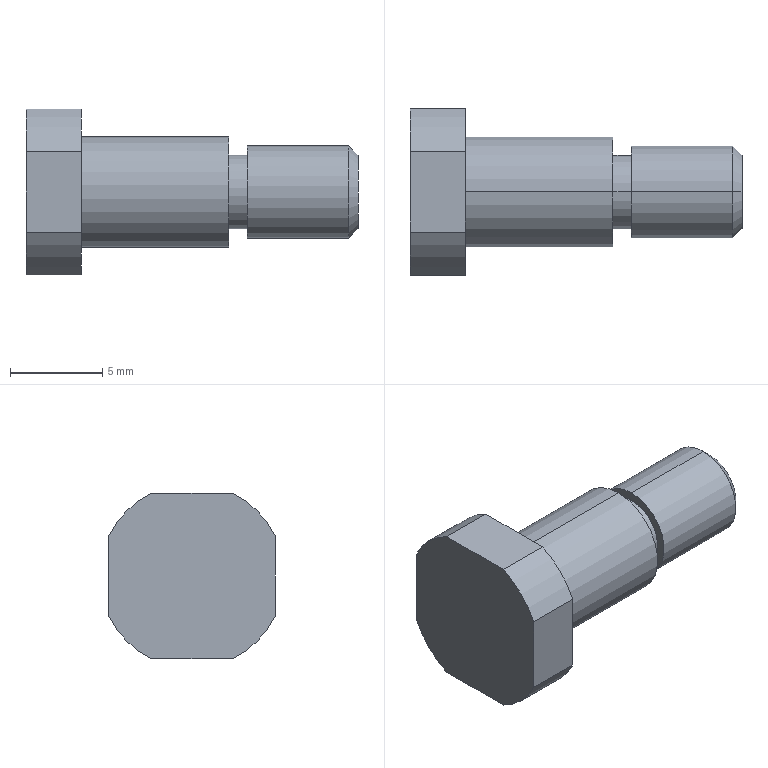Component | SolidWorks | A51-3 | 1 solid | 21 faces | box 18 x 9 x 9 mm | volume 573 mm3 | cylinder 10 | plane 9 | cone 2 | commonest cylinder face diameters 10 x4 5 x2 4 x2 6 x2 | material SUS304
build123d program:
from build123d import *

# Parameters (mm, degrees)
SKETCH12_R           = 5
BOSS_EXTRUDE3_DEPTH  = 3
SKETCH13_R           = 3
BOSS_EXTRUDE4_DEPTH  = 8
SKETCH14_R           = 2
BOSS_EXTRUDE5_DEPTH  = 1
SKETCH15_R           = 2.5
BOSS_EXTRUDE6_DEPTH  = 6
CHAMFER4_SIZE        = 0.5
SKETCH16_OUTSIDE_W   = 16.578
SKETCH16_OUTSIDE_H   = 16.578
SKETCH16_OUTSIDE_W_2 = 9
SKETCH16_OUTSIDE_H_2 = 9
CUT_EXTRUDE1_DEPTH   = 20.339


with BuildPart() as part:
    # Sketch12 → Boss-Extrude3 (new body)
    with BuildSketch(Plane(origin=(0, 0, 0), x_dir=(0, 0, -1), z_dir=(1, 0, 0))):
        Circle(SKETCH12_R)
    extrude(amount=BOSS_EXTRUDE3_DEPTH)

    # Sketch13 → Boss-Extrude4 (add)
    with BuildSketch(Plane.ZY):
        Circle(SKETCH13_R)
    extrude(amount=BOSS_EXTRUDE4_DEPTH)

    # Sketch14 → Boss-Extrude5 (add)
    with BuildSketch(Plane.ZY.offset(8)):
        Circle(SKETCH14_R)
    extrude(amount=BOSS_EXTRUDE5_DEPTH)

    # Sketch15 → Boss-Extrude6 (add)
    with BuildSketch(Plane.ZY.offset(9)):
        Circle(SKETCH15_R)
    extrude(amount=BOSS_EXTRUDE6_DEPTH)

    # Chamfer4
    chamfer4_edges = [part.edges().sort_by_distance(p)[0] for p in [
        (-15, 0, -2.5),
    ]]
    chamfer(chamfer4_edges, length=CHAMFER4_SIZE)

    # Sketch16 outside → Cut-Extrude1 (cut, through all)
    with BuildSketch(Plane(origin=(3, 0, 0), x_dir=(0, 0, -1), z_dir=(1, 0, 0))):
        Rectangle(SKETCH16_OUTSIDE_W, SKETCH16_OUTSIDE_H)
        Rectangle(SKETCH16_OUTSIDE_W_2, SKETCH16_OUTSIDE_H_2, mode=Mode.SUBTRACT)
    extrude(amount=-CUT_EXTRUDE1_DEPTH, mode=Mode.SUBTRACT)


solid = part.part

# Placed as in the assembly
solid = solid.moved(Location((-25.351, 25.864, 5), (-180, 0, 180)))
STEP:
#1=CARTESIAN_POINT('',(-0.4075,1.018,0.1181));
#2=VERTEX_POINT('',#1);
#3=CARTESIAN_POINT('',(-0.4075,1.018,0.2756));
#4=VERTEX_POINT('',#3);
#5=CARTESIAN_POINT('',(-0.4075,1.018,0.1969));
#6=DIRECTION('',(1.,0.,0.));
#7=DIRECTION('',(0.,0.,-1.));
#8=AXIS2_PLACEMENT_3D('',#5,#6,#7);
#9=CIRCLE('',#8,0.07874);
#10=EDGE_CURVE('',#2,#4,#9,.T.);
#11=ORIENTED_EDGE('',*,*,#10,.F.);
#12=CARTESIAN_POINT('',(-0.4272,1.018,0.09843));
#13=VERTEX_POINT('',#12);
#14=CARTESIAN_POINT('',(-0.4075,1.018,0.1181));
#15=DIRECTION('',(-0.7071,0.,-0.7071));
#16=VECTOR('',#15,39.37);
#17=LINE('',#14,#16);
#18=EDGE_CURVE('',#2,#13,#17,.T.);
#19=ORIENTED_EDGE('',*,*,#18,.T.);
#20=CARTESIAN_POINT('',(-0.4272,1.018,0.2953));
#21=VERTEX_POINT('',#20);
#22=CARTESIAN_POINT('',(-0.4272,1.018,0.1969));
#23=DIRECTION('',(-1.,-0.,-0.));
#24=DIRECTION('',(0.,0.,-1.));
#25=AXIS2_PLACEMENT_3D('',#22,#23,#24);
#26=CIRCLE('',#25,0.09843);
#27=EDGE_CURVE('',#21,#13,#26,.T.);
#28=ORIENTED_EDGE('',*,*,#27,.F.);
#29=CARTESIAN_POINT('',(-0.4075,1.018,0.2756));
#30=DIRECTION('',(-0.7071,-0.,0.7071));
#31=VECTOR('',#30,39.37);
#32=LINE('',#29,#31);
#33=EDGE_CURVE('',#4,#21,#32,.T.);
#34=ORIENTED_EDGE('',*,*,#33,.F.);
#35=EDGE_LOOP('',(#11,#19,#28,#34));
#36=FACE_OUTER_BOUND('',#35,.T.);
#37=CARTESIAN_POINT('',(-0.4075,1.018,0.1969));
#38=DIRECTION('',(-1.,-0.,-0.));
#39=DIRECTION('',(0.,0.,1.));
#40=AXIS2_PLACEMENT_3D('',#37,#38,#39);
#41=CONICAL_SURFACE('',#40,0.07874,0.7854);
#42=ADVANCED_FACE('',(#36),#41,.T.);
#43=ORIENTED_EDGE('',*,*,#27,.T.);
#44=CARTESIAN_POINT('',(-0.6437,1.018,0.09843));
#45=VERTEX_POINT('',#44);
#46=CARTESIAN_POINT('',(-0.4075,1.018,0.09843));
#47=DIRECTION('',(-1.,-0.,-0.));
#48=VECTOR('',#47,39.37);
#49=LINE('',#46,#48);
#50=EDGE_CURVE('',#13,#45,#49,.T.);
#51=ORIENTED_EDGE('',*,*,#50,.T.);
#52=CARTESIAN_POINT('',(-0.6437,1.018,0.2953));
#53=VERTEX_POINT('',#52);
#54=CARTESIAN_POINT('',(-0.6437,1.018,0.1969));
#55=DIRECTION('',(1.,0.,0.));
#56=DIRECTION('',(0.,0.,-1.));
#57=AXIS2_PLACEMENT_3D('',#54,#55,#56);
#58=CIRCLE('',#57,0.09843);
#59=EDGE_CURVE('',#45,#53,#58,.T.);
#60=ORIENTED_EDGE('',*,*,#59,.T.);
#61=CARTESIAN_POINT('',(-0.4075,1.018,0.2953));
#62=DIRECTION('',(-1.,-0.,-0.));
#63=VECTOR('',#62,39.37);
#64=LINE('',#61,#63);
#65=EDGE_CURVE('',#21,#53,#64,.T.);
#66=ORIENTED_EDGE('',*,*,#65,.F.);
#67=EDGE_LOOP('',(#43,#51,#60,#66));
#68=FACE_OUTER_BOUND('',#67,.T.);
#69=CARTESIAN_POINT('',(-0.4075,1.018,0.1969));
#70=DIRECTION('',(-1.,-0.,-0.));
#71=DIRECTION('',(0.,0.,1.));
#72=AXIS2_PLACEMENT_3D('',#69,#70,#71);
#73=CYLINDRICAL_SURFACE('',#72,0.09843);
#74=ADVANCED_FACE('',(#68),#73,.T.);
#75=CARTESIAN_POINT('',(-0.6437,1.018,0.1181));
#76=VERTEX_POINT('',#75);
#77=CARTESIAN_POINT('',(-0.6437,1.018,0.2756));
#78=VERTEX_POINT('',#77);
#79=CARTESIAN_POINT('',(-0.6437,1.018,0.1969));
#80=DIRECTION('',(1.,0.,0.));
#81=DIRECTION('',(0.,0.,-1.));
#82=AXIS2_PLACEMENT_3D('',#79,#80,#81);
#83=CIRCLE('',#82,0.07874);
#84=EDGE_CURVE('',#76,#78,#83,.T.);
#85=ORIENTED_EDGE('',*,*,#84,.F.);
#86=CARTESIAN_POINT('',(-0.6831,1.018,0.1181));
#87=VERTEX_POINT('',#86);
#88=CARTESIAN_POINT('',(-0.6437,1.018,0.1181));
#89=DIRECTION('',(-1.,-0.,-0.));
#90=VECTOR('',#89,39.37);
#91=LINE('',#88,#90);
#92=EDGE_CURVE('',#76,#87,#91,.T.);
#93=ORIENTED_EDGE('',*,*,#92,.T.);
#94=CARTESIAN_POINT('',(-0.6831,1.018,0.2756));
#95=VERTEX_POINT('',#94);
#96=CARTESIAN_POINT('',(-0.6831,1.018,0.1969));
#97=DIRECTION('',(1.,0.,0.));
#98=DIRECTION('',(0.,0.,-1.));
#99=AXIS2_PLACEMENT_3D('',#96,#97,#98);
#100=CIRCLE('',#99,0.07874);
#101=EDGE_CURVE('',#87,#95,#100,.T.);
#102=ORIENTED_EDGE('',*,*,#101,.T.);
#103=CARTESIAN_POINT('',(-0.6437,1.018,0.2756));
#104=DIRECTION('',(-1.,-0.,-0.));
#105=VECTOR('',#104,39.37);
#106=LINE('',#103,#105);
#107=EDGE_CURVE('',#78,#95,#106,.T.);
#108=ORIENTED_EDGE('',*,*,#107,.F.);
#109=EDGE_LOOP('',(#85,#93,#102,#108));
#110=FACE_OUTER_BOUND('',#109,.T.);
#111=CARTESIAN_POINT('',(-0.6437,1.018,0.1969));
#112=DIRECTION('',(-1.,-0.,-0.));
#113=DIRECTION('',(0.,0.,1.));
#114=AXIS2_PLACEMENT_3D('',#111,#112,#113);
#115=CYLINDRICAL_SURFACE('',#114,0.07874);
#116=ADVANCED_FACE('',(#110),#115,.T.);
#117=CARTESIAN_POINT('',(-0.6831,1.018,0.07874));
#118=VERTEX_POINT('',#117);
#119=CARTESIAN_POINT('',(-0.6831,1.018,0.315));
#120=VERTEX_POINT('',#119);
#121=CARTESIAN_POINT('',(-0.6831,1.018,0.1969));
#122=DIRECTION('',(1.,0.,0.));
#123=DIRECTION('',(0.,0.,-1.));
#124=AXIS2_PLACEMENT_3D('',#121,#122,#123);
#125=CIRCLE('',#124,0.1181);
#126=EDGE_CURVE('',#118,#120,#125,.T.);
#127=ORIENTED_EDGE('',*,*,#126,.F.);
#128=CARTESIAN_POINT('',(-0.9981,1.018,0.07874));
#129=VERTEX_POINT('',#128);
#130=CARTESIAN_POINT('',(-0.6831,1.018,0.07874));
#131=DIRECTION('',(-1.,-0.,-0.));
#132=VECTOR('',#131,39.37);
#133=LINE('',#130,#132);
#134=EDGE_CURVE('',#118,#129,#133,.T.);
#135=ORIENTED_EDGE('',*,*,#134,.T.);
#136=CARTESIAN_POINT('',(-0.9981,1.018,0.315));
#137=VERTEX_POINT('',#136);
#138=CARTESIAN_POINT('',(-0.9981,1.018,0.1969));
#139=DIRECTION('',(1.,0.,0.));
#140=DIRECTION('',(0.,0.,-1.));
#141=AXIS2_PLACEMENT_3D('',#138,#139,#140);
#142=CIRCLE('',#141,0.1181);
#143=EDGE_CURVE('',#129,#137,#142,.T.);
#144=ORIENTED_EDGE('',*,*,#143,.T.);
#145=CARTESIAN_POINT('',(-0.6831,1.018,0.315));
#146=DIRECTION('',(-1.,-0.,-0.));
#147=VECTOR('',#146,39.37);
#148=LINE('',#145,#147);
#149=EDGE_CURVE('',#120,#137,#148,.T.);
#150=ORIENTED_EDGE('',*,*,#149,.F.);
#151=EDGE_LOOP('',(#127,#135,#144,#150));
#152=FACE_OUTER_BOUND('',#151,.T.);
#153=CARTESIAN_POINT('',(-0.6831,1.018,0.1969));
#154=DIRECTION('',(-1.,-0.,-0.));
#155=DIRECTION('',(0.,0.,1.));
#156=AXIS2_PLACEMENT_3D('',#153,#154,#155);
#157=CYLINDRICAL_SURFACE('',#156,0.1181);
#158=ADVANCED_FACE('',(#152),#157,.T.);
#159=CARTESIAN_POINT('',(-1.116,0.9325,0.374));
#160=VERTEX_POINT('',#159);
#161=CARTESIAN_POINT('',(-0.9981,0.9325,0.374));
#162=VERTEX_POINT('',#161);
#163=CARTESIAN_POINT('',(-1.116,0.9325,0.374));
#164=DIRECTION('',(1.,0.,0.));
#165=VECTOR('',#164,39.37);
#166=LINE('',#163,#165);
#167=EDGE_CURVE('',#160,#162,#166,.T.);
#168=ORIENTED_EDGE('',*,*,#167,.F.);
#169=CARTESIAN_POINT('',(-1.116,0.8411,0.2827));
#170=VERTEX_POINT('',#169);
#171=CARTESIAN_POINT('',(-1.116,1.018,0.1969));
#172=DIRECTION('',(-1.,-0.,-0.));
#173=DIRECTION('',(0.,0.,1.));
#174=AXIS2_PLACEMENT_3D('',#171,#172,#173);
#175=CIRCLE('',#174,0.1969);
#176=EDGE_CURVE('',#170,#160,#175,.T.);
#177=ORIENTED_EDGE('',*,*,#176,.F.);
#178=CARTESIAN_POINT('',(-0.9981,0.8411,0.2827));
#179=VERTEX_POINT('',#178);
#180=CARTESIAN_POINT('',(-1.116,0.8411,0.2827));
#181=DIRECTION('',(-1.,-0.,-0.));
#182=VECTOR('',#181,39.37);
#183=LINE('',#180,#182);
#184=EDGE_CURVE('',#179,#170,#183,.T.);
#185=ORIENTED_EDGE('',*,*,#184,.F.);
#186=CARTESIAN_POINT('',(-0.9981,1.018,0.1969));
#187=DIRECTION('',(-1.,-0.,-0.));
#188=DIRECTION('',(0.,0.,1.));
#189=AXIS2_PLACEMENT_3D('',#186,#187,#188);
#190=CIRCLE('',#189,0.1969);
#191=EDGE_CURVE('',#179,#162,#190,.T.);
#192=ORIENTED_EDGE('',*,*,#191,.T.);
#193=EDGE_LOOP('',(#168,#177,#185,#192));
#194=FACE_OUTER_BOUND('',#193,.T.);
#195=CARTESIAN_POINT('',(-1.116,1.018,0.1969));
#196=DIRECTION('',(1.,0.,0.));
#197=DIRECTION('',(0.,0.,-1.));
#198=AXIS2_PLACEMENT_3D('',#195,#196,#197);
#199=CYLINDRICAL_SURFACE('',#198,0.1969);
#200=ADVANCED_FACE('',(#194),#199,.T.);
#201=CARTESIAN_POINT('',(-0.9981,1.104,0.374));
#202=VERTEX_POINT('',#201);
#203=CARTESIAN_POINT('',(-1.116,1.104,0.374));
#204=VERTEX_POINT('',#203);
#205=CARTESIAN_POINT('',(-1.116,1.104,0.374));
#206=DIRECTION('',(-1.,-0.,-0.));
#207=VECTOR('',#206,39.37);
#208=LINE('',#205,#207);
#209=EDGE_CURVE('',#202,#204,#208,.T.);
#210=ORIENTED_EDGE('',*,*,#209,.F.);
#211=CARTESIAN_POINT('',(-0.9981,1.195,0.2827));
#212=VERTEX_POINT('',#211);
#213=CARTESIAN_POINT('',(-0.9981,1.018,0.1969));
#214=DIRECTION('',(-1.,-0.,-0.));
#215=DIRECTION('',(0.,0.,1.));
#216=AXIS2_PLACEMENT_3D('',#213,#214,#215);
#217=CIRCLE('',#216,0.1969);
#218=EDGE_CURVE('',#202,#212,#217,.T.);
#219=ORIENTED_EDGE('',*,*,#218,.T.);
#220=CARTESIAN_POINT('',(-1.116,1.195,0.2827));
#221=VERTEX_POINT('',#220);
#222=CARTESIAN_POINT('',(-1.116,1.195,0.2827));
#223=DIRECTION('',(1.,0.,0.));
#224=VECTOR('',#223,39.37);
#225=LINE('',#222,#224);
#226=EDGE_CURVE('',#221,#212,#225,.T.);
#227=ORIENTED_EDGE('',*,*,#226,.F.);
#228=CARTESIAN_POINT('',(-1.116,1.018,0.1969));
#229=DIRECTION('',(-1.,-0.,-0.));
#230=DIRECTION('',(0.,0.,1.));
#231=AXIS2_PLACEMENT_3D('',#228,#229,#230);
#232=CIRCLE('',#231,0.1969);
#233=EDGE_CURVE('',#204,#221,#232,.T.);
#234=ORIENTED_EDGE('',*,*,#233,.F.);
#235=EDGE_LOOP('',(#210,#219,#227,#234));
#236=FACE_OUTER_BOUND('',#235,.T.);
#237=CARTESIAN_POINT('',(-1.116,1.018,0.1969));
#238=DIRECTION('',(1.,0.,0.));
#239=DIRECTION('',(0.,0.,-1.));
#240=AXIS2_PLACEMENT_3D('',#237,#238,#239);
#241=CYLINDRICAL_SURFACE('',#240,0.1969);
#242=ADVANCED_FACE('',(#236),#241,.T.);
#243=CARTESIAN_POINT('',(-1.116,0.8411,0.111));
#244=VERTEX_POINT('',#243);
#245=CARTESIAN_POINT('',(-0.9981,0.8411,0.111));
#246=VERTEX_POINT('',#245);
#247=CARTESIAN_POINT('',(-1.116,0.8411,0.111));
#248=DIRECTION('',(1.,0.,0.));
#249=VECTOR('',#248,39.37);
#250=LINE('',#247,#249);
#251=EDGE_CURVE('',#244,#246,#250,.T.);
#252=ORIENTED_EDGE('',*,*,#251,.F.);
#253=CARTESIAN_POINT('',(-1.116,0.9325,0.01969));
#254=VERTEX_POINT('',#253);
#255=CARTESIAN_POINT('',(-1.116,1.018,0.1969));
#256=DIRECTION('',(-1.,-0.,-0.));
#257=DIRECTION('',(0.,0.,1.));
#258=AXIS2_PLACEMENT_3D('',#255,#256,#257);
#259=CIRCLE('',#258,0.1969);
#260=EDGE_CURVE('',#254,#244,#259,.T.);
#261=ORIENTED_EDGE('',*,*,#260,.F.);
#262=CARTESIAN_POINT('',(-0.9981,0.9325,0.01969));
#263=VERTEX_POINT('',#262);
#264=CARTESIAN_POINT('',(-1.116,0.9325,0.01969));
#265=DIRECTION('',(-1.,-0.,-0.));
#266=VECTOR('',#265,39.37);
#267=LINE('',#264,#266);
#268=EDGE_CURVE('',#263,#254,#267,.T.);
#269=ORIENTED_EDGE('',*,*,#268,.F.);
#270=CARTESIAN_POINT('',(-0.9981,1.018,0.1969));
#271=DIRECTION('',(-1.,-0.,-0.));
#272=DIRECTION('',(0.,0.,1.));
#273=AXIS2_PLACEMENT_3D('',#270,#271,#272);
#274=CIRCLE('',#273,0.1969);
#275=EDGE_CURVE('',#263,#246,#274,.T.);
#276=ORIENTED_EDGE('',*,*,#275,.T.);
#277=EDGE_LOOP('',(#252,#261,#269,#276));
#278=FACE_OUTER_BOUND('',#277,.T.);
#279=CARTESIAN_POINT('',(-1.116,1.018,0.1969));
#280=DIRECTION('',(1.,0.,0.));
#281=DIRECTION('',(0.,0.,-1.));
#282=AXIS2_PLACEMENT_3D('',#279,#280,#281);
#283=CYLINDRICAL_SURFACE('',#282,0.1969);
#284=ADVANCED_FACE('',(#278),#283,.T.);
#285=CARTESIAN_POINT('',(-1.116,1.104,0.01969));
#286=VERTEX_POINT('',#285);
#287=CARTESIAN_POINT('',(-0.9981,1.104,0.01969));
#288=VERTEX_POINT('',#287);
#289=CARTESIAN_POINT('',(-1.116,1.104,0.01969));
#290=DIRECTION('',(1.,0.,0.));
#291=VECTOR('',#290,39.37);
#292=LINE('',#289,#291);
#293=EDGE_CURVE('',#286,#288,#292,.T.);
#294=ORIENTED_EDGE('',*,*,#293,.F.);
#295=CARTESIAN_POINT('',(-1.116,1.195,0.111));
#296=VERTEX_POINT('',#295);
#297=CARTESIAN_POINT('',(-1.116,1.018,0.1969));
#298=DIRECTION('',(-1.,-0.,-0.));
#299=DIRECTION('',(0.,0.,1.));
#300=AXIS2_PLACEMENT_3D('',#297,#298,#299);
#301=CIRCLE('',#300,0.1969);
#302=EDGE_CURVE('',#296,#286,#301,.T.);
#303=ORIENTED_EDGE('',*,*,#302,.F.);
#304=CARTESIAN_POINT('',(-0.9981,1.195,0.111));
#305=VERTEX_POINT('',#304);
#306=CARTESIAN_POINT('',(-1.116,1.195,0.111));
#307=DIRECTION('',(-1.,-0.,-0.));
#308=VECTOR('',#307,39.37);
#309=LINE('',#306,#308);
#310=EDGE_CURVE('',#305,#296,#309,.T.);
#311=ORIENTED_EDGE('',*,*,#310,.F.);
#312=CARTESIAN_POINT('',(-0.9981,1.018,0.1969));
#313=DIRECTION('',(-1.,-0.,-0.));
#314=DIRECTION('',(0.,0.,1.));
#315=AXIS2_PLACEMENT_3D('',#312,#313,#314);
#316=CIRCLE('',#315,0.1969);
#317=EDGE_CURVE('',#305,#288,#316,.T.);
#318=ORIENTED_EDGE('',*,*,#317,.T.);
#319=EDGE_LOOP('',(#294,#303,#311,#318));
#320=FACE_OUTER_BOUND('',#319,.T.);
#321=CARTESIAN_POINT('',(-1.116,1.018,0.1969));
#322=DIRECTION('',(1.,0.,0.));
#323=DIRECTION('',(0.,0.,-1.));
#324=AXIS2_PLACEMENT_3D('',#321,#322,#323);
#325=CYLINDRICAL_SURFACE('',#324,0.1969);
#326=ADVANCED_FACE('',(#320),#325,.T.);
#327=ORIENTED_EDGE('',*,*,#176,.T.);
#328=CARTESIAN_POINT('',(-1.116,1.195,0.374));
#329=DIRECTION('',(-0.,1.,0.));
#330=VECTOR('',#329,39.37);
#331=LINE('',#328,#330);
#332=EDGE_CURVE('',#160,#204,#331,.T.);
#333=ORIENTED_EDGE('',*,*,#332,.T.);
#334=ORIENTED_EDGE('',*,*,#233,.T.);
#335=CARTESIAN_POINT('',(-1.116,1.195,0.01969));
#336=DIRECTION('',(0.,0.,-1.));
#337=VECTOR('',#336,39.37);
#338=LINE('',#335,#337);
#339=EDGE_CURVE('',#221,#296,#338,.T.);
#340=ORIENTED_EDGE('',*,*,#339,.T.);
#341=ORIENTED_EDGE('',*,*,#302,.T.);
#342=CARTESIAN_POINT('',(-1.116,1.195,0.01969));
#343=DIRECTION('',(0.,-1.,-0.));
#344=VECTOR('',#343,39.37);
#345=LINE('',#342,#344);
#346=EDGE_CURVE('',#286,#254,#345,.T.);
#347=ORIENTED_EDGE('',*,*,#346,.T.);
#348=ORIENTED_EDGE('',*,*,#260,.T.);
#349=CARTESIAN_POINT('',(-1.116,0.8411,0.01969));
#350=DIRECTION('',(-0.,-0.,1.));
#351=VECTOR('',#350,39.37);
#352=LINE('',#349,#351);
#353=EDGE_CURVE('',#244,#170,#352,.T.);
#354=ORIENTED_EDGE('',*,*,#353,.T.);
#355=EDGE_LOOP('',(#327,#333,#334,#340,#341,#347,#348,#354));
#356=FACE_OUTER_BOUND('',#355,.T.);
#357=CARTESIAN_POINT('',(-1.116,1.018,0.1969));
#358=DIRECTION('',(-1.,-0.,-0.));
#359=DIRECTION('',(-0.,-0.,1.));
#360=AXIS2_PLACEMENT_3D('',#357,#358,#359);
#361=PLANE('',#360);
#362=ADVANCED_FACE('',(#356),#361,.T.);
#363=CARTESIAN_POINT('',(-0.9981,1.018,0.1969));
#364=DIRECTION('',(1.,0.,0.));
#365=DIRECTION('',(0.,0.,-1.));
#366=AXIS2_PLACEMENT_3D('',#363,#364,#365);
#367=CIRCLE('',#366,0.1181);
#368=EDGE_CURVE('',#137,#129,#367,.T.);
#369=ORIENTED_EDGE('',*,*,#368,.F.);
#370=ORIENTED_EDGE('',*,*,#143,.F.);
#371=EDGE_LOOP('',(#369,#370));
#372=FACE_BOUND('',#371,.T.);
#373=CARTESIAN_POINT('',(-0.9981,1.018,0.374));
#374=DIRECTION('',(-0.,1.,0.));
#375=VECTOR('',#374,39.37);
#376=LINE('',#373,#375);
#377=EDGE_CURVE('',#162,#202,#376,.T.);
#378=ORIENTED_EDGE('',*,*,#377,.F.);
#379=ORIENTED_EDGE('',*,*,#191,.F.);
#380=CARTESIAN_POINT('',(-0.9981,0.8411,0.1969));
#381=DIRECTION('',(-0.,-0.,1.));
#382=VECTOR('',#381,39.37);
#383=LINE('',#380,#382);
#384=EDGE_CURVE('',#246,#179,#383,.T.);
#385=ORIENTED_EDGE('',*,*,#384,.F.);
#386=ORIENTED_EDGE('',*,*,#275,.F.);
#387=CARTESIAN_POINT('',(-0.9981,1.018,0.01969));
#388=DIRECTION('',(0.,-1.,-0.));
#389=VECTOR('',#388,39.37);
#390=LINE('',#387,#389);
#391=EDGE_CURVE('',#288,#263,#390,.T.);
#392=ORIENTED_EDGE('',*,*,#391,.F.);
#393=ORIENTED_EDGE('',*,*,#317,.F.);
#394=CARTESIAN_POINT('',(-0.9981,1.195,0.1969));
#395=DIRECTION('',(0.,0.,-1.));
#396=VECTOR('',#395,39.37);
#397=LINE('',#394,#396);
#398=EDGE_CURVE('',#212,#305,#397,.T.);
#399=ORIENTED_EDGE('',*,*,#398,.F.);
#400=ORIENTED_EDGE('',*,*,#218,.F.);
#401=EDGE_LOOP('',(#378,#379,#385,#386,#392,#393,#399,#400));
#402=FACE_OUTER_BOUND('',#401,.T.);
#403=CARTESIAN_POINT('',(-0.9981,1.018,0.1969));
#404=DIRECTION('',(-1.,-0.,-0.));
#405=DIRECTION('',(-0.,-0.,1.));
#406=AXIS2_PLACEMENT_3D('',#403,#404,#405);
#407=PLANE('',#406);
#408=ADVANCED_FACE('',(#372,#402),#407,.F.);
#409=ORIENTED_EDGE('',*,*,#134,.F.);
#410=CARTESIAN_POINT('',(-0.6831,1.018,0.1969));
#411=DIRECTION('',(1.,0.,0.));
#412=DIRECTION('',(0.,0.,-1.));
#413=AXIS2_PLACEMENT_3D('',#410,#411,#412);
#414=CIRCLE('',#413,0.1181);
#415=EDGE_CURVE('',#120,#118,#414,.T.);
#416=ORIENTED_EDGE('',*,*,#415,.F.);
#417=ORIENTED_EDGE('',*,*,#149,.T.);
#418=ORIENTED_EDGE('',*,*,#368,.T.);
#419=EDGE_LOOP('',(#409,#416,#417,#418));
#420=FACE_OUTER_BOUND('',#419,.T.);
#421=CARTESIAN_POINT('',(-0.6831,1.018,0.1969));
#422=DIRECTION('',(-1.,-0.,-0.));
#423=DIRECTION('',(0.,0.,1.));
#424=AXIS2_PLACEMENT_3D('',#421,#422,#423);
#425=CYLINDRICAL_SURFACE('',#424,0.1181);
#426=ADVANCED_FACE('',(#420),#425,.T.);
#427=CARTESIAN_POINT('',(-0.6831,1.018,0.1969));
#428=DIRECTION('',(1.,0.,0.));
#429=DIRECTION('',(0.,0.,-1.));
#430=AXIS2_PLACEMENT_3D('',#427,#428,#429);
#431=CIRCLE('',#430,0.07874);
#432=EDGE_CURVE('',#95,#87,#431,.T.);
#433=ORIENTED_EDGE('',*,*,#432,.F.);
#434=ORIENTED_EDGE('',*,*,#101,.F.);
#435=EDGE_LOOP('',(#433,#434));
#436=FACE_BOUND('',#435,.T.);
#437=ORIENTED_EDGE('',*,*,#415,.T.);
#438=ORIENTED_EDGE('',*,*,#126,.T.);
#439=EDGE_LOOP('',(#437,#438));
#440=FACE_OUTER_BOUND('',#439,.T.);
#441=CARTESIAN_POINT('',(-0.6831,1.018,0.1969));
#442=DIRECTION('',(1.,0.,0.));
#443=DIRECTION('',(0.,0.,-1.));
#444=AXIS2_PLACEMENT_3D('',#441,#442,#443);
#445=PLANE('',#444);
#446=ADVANCED_FACE('',(#436,#440),#445,.T.);
#447=ORIENTED_EDGE('',*,*,#92,.F.);
#448=CARTESIAN_POINT('',(-0.6437,1.018,0.1969));
#449=DIRECTION('',(1.,0.,0.));
#450=DIRECTION('',(0.,0.,-1.));
#451=AXIS2_PLACEMENT_3D('',#448,#449,#450);
#452=CIRCLE('',#451,0.07874);
#453=EDGE_CURVE('',#78,#76,#452,.T.);
#454=ORIENTED_EDGE('',*,*,#453,.F.);
#455=ORIENTED_EDGE('',*,*,#107,.T.);
#456=ORIENTED_EDGE('',*,*,#432,.T.);
#457=EDGE_LOOP('',(#447,#454,#455,#456));
#458=FACE_OUTER_BOUND('',#457,.T.);
#459=CARTESIAN_POINT('',(-0.6437,1.018,0.1969));
#460=DIRECTION('',(-1.,-0.,-0.));
#461=DIRECTION('',(0.,0.,1.));
#462=AXIS2_PLACEMENT_3D('',#459,#460,#461);
#463=CYLINDRICAL_SURFACE('',#462,0.07874);
#464=ADVANCED_FACE('',(#458),#463,.T.);
#465=ORIENTED_EDGE('',*,*,#50,.F.);
#466=CARTESIAN_POINT('',(-0.4272,1.018,0.1969));
#467=DIRECTION('',(-1.,-0.,-0.));
#468=DIRECTION('',(0.,0.,-1.));
#469=AXIS2_PLACEMENT_3D('',#466,#467,#468);
#470=CIRCLE('',#469,0.09843);
#471=EDGE_CURVE('',#13,#21,#470,.T.);
#472=ORIENTED_EDGE('',*,*,#471,.T.);
#473=ORIENTED_EDGE('',*,*,#65,.T.);
#474=CARTESIAN_POINT('',(-0.6437,1.018,0.1969));
#475=DIRECTION('',(1.,0.,0.));
#476=DIRECTION('',(0.,0.,-1.));
#477=AXIS2_PLACEMENT_3D('',#474,#475,#476);
#478=CIRCLE('',#477,0.09843);
#479=EDGE_CURVE('',#53,#45,#478,.T.);
#480=ORIENTED_EDGE('',*,*,#479,.T.);
#481=EDGE_LOOP('',(#465,#472,#473,#480));
#482=FACE_OUTER_BOUND('',#481,.T.);
#483=CARTESIAN_POINT('',(-0.4075,1.018,0.1969));
#484=DIRECTION('',(-1.,-0.,-0.));
#485=DIRECTION('',(0.,0.,1.));
#486=AXIS2_PLACEMENT_3D('',#483,#484,#485);
#487=CYLINDRICAL_SURFACE('',#486,0.09843);
#488=ADVANCED_FACE('',(#482),#487,.T.);
#489=CARTESIAN_POINT('',(-0.4075,1.018,0.1969));
#490=DIRECTION('',(1.,0.,0.));
#491=DIRECTION('',(0.,0.,-1.));
#492=AXIS2_PLACEMENT_3D('',#489,#490,#491);
#493=CIRCLE('',#492,0.07874);
#494=EDGE_CURVE('',#4,#2,#493,.T.);
#495=ORIENTED_EDGE('',*,*,#494,.T.);
#496=ORIENTED_EDGE('',*,*,#10,.T.);
#497=EDGE_LOOP('',(#495,#496));
#498=FACE_OUTER_BOUND('',#497,.T.);
#499=CARTESIAN_POINT('',(-0.4075,1.018,0.1969));
#500=DIRECTION('',(1.,0.,0.));
#501=DIRECTION('',(0.,0.,-1.));
#502=AXIS2_PLACEMENT_3D('',#499,#500,#501);
#503=PLANE('',#502);
#504=ADVANCED_FACE('',(#498),#503,.T.);
#505=ORIENTED_EDGE('',*,*,#453,.T.);
#506=ORIENTED_EDGE('',*,*,#84,.T.);
#507=EDGE_LOOP('',(#505,#506));
#508=FACE_BOUND('',#507,.T.);
#509=ORIENTED_EDGE('',*,*,#479,.F.);
#510=ORIENTED_EDGE('',*,*,#59,.F.);
#511=EDGE_LOOP('',(#509,#510));
#512=FACE_OUTER_BOUND('',#511,.T.);
#513=CARTESIAN_POINT('',(-0.6437,1.018,0.1969));
#514=DIRECTION('',(1.,0.,0.));
#515=DIRECTION('',(0.,0.,-1.));
#516=AXIS2_PLACEMENT_3D('',#513,#514,#515);
#517=PLANE('',#516);
#518=ADVANCED_FACE('',(#508,#512),#517,.F.);
#519=ORIENTED_EDGE('',*,*,#18,.F.);
#520=ORIENTED_EDGE('',*,*,#494,.F.);
#521=ORIENTED_EDGE('',*,*,#33,.T.);
#522=ORIENTED_EDGE('',*,*,#471,.F.);
#523=EDGE_LOOP('',(#519,#520,#521,#522));
#524=FACE_OUTER_BOUND('',#523,.T.);
#525=CARTESIAN_POINT('',(-0.4075,1.018,0.1969));
#526=DIRECTION('',(-1.,-0.,-0.));
#527=DIRECTION('',(0.,0.,1.));
#528=AXIS2_PLACEMENT_3D('',#525,#526,#527);
#529=CONICAL_SURFACE('',#528,0.07874,0.7854);
#530=ADVANCED_FACE('',(#524),#529,.T.);
#531=ORIENTED_EDGE('',*,*,#226,.T.);
#532=ORIENTED_EDGE('',*,*,#398,.T.);
#533=ORIENTED_EDGE('',*,*,#310,.T.);
#534=ORIENTED_EDGE('',*,*,#339,.F.);
#535=EDGE_LOOP('',(#531,#532,#533,#534));
#536=FACE_OUTER_BOUND('',#535,.T.);
#537=CARTESIAN_POINT('',(-0.4075,1.195,0.01969));
#538=DIRECTION('',(-0.,1.,0.));
#539=DIRECTION('',(0.,0.,-1.));
#540=AXIS2_PLACEMENT_3D('',#537,#538,#539);
#541=PLANE('',#540);
#542=ADVANCED_FACE('',(#536),#541,.T.);
#543=ORIENTED_EDGE('',*,*,#293,.T.);
#544=ORIENTED_EDGE('',*,*,#391,.T.);
#545=ORIENTED_EDGE('',*,*,#268,.T.);
#546=ORIENTED_EDGE('',*,*,#346,.F.);
#547=EDGE_LOOP('',(#543,#544,#545,#546));
#548=FACE_OUTER_BOUND('',#547,.T.);
#549=CARTESIAN_POINT('',(-0.4075,1.195,0.01969));
#550=DIRECTION('',(0.,0.,-1.));
#551=DIRECTION('',(-1.,-0.,-0.));
#552=AXIS2_PLACEMENT_3D('',#549,#550,#551);
#553=PLANE('',#552);
#554=ADVANCED_FACE('',(#548),#553,.T.);
#555=ORIENTED_EDGE('',*,*,#251,.T.);
#556=ORIENTED_EDGE('',*,*,#384,.T.);
#557=ORIENTED_EDGE('',*,*,#184,.T.);
#558=ORIENTED_EDGE('',*,*,#353,.F.);
#559=EDGE_LOOP('',(#555,#556,#557,#558));
#560=FACE_OUTER_BOUND('',#559,.T.);
#561=CARTESIAN_POINT('',(-0.4075,0.8411,0.01969));
#562=DIRECTION('',(0.,-1.,-0.));
#563=DIRECTION('',(-0.,-0.,1.));
#564=AXIS2_PLACEMENT_3D('',#561,#562,#563);
#565=PLANE('',#564);
#566=ADVANCED_FACE('',(#560),#565,.T.);
#567=ORIENTED_EDGE('',*,*,#167,.T.);
#568=ORIENTED_EDGE('',*,*,#377,.T.);
#569=ORIENTED_EDGE('',*,*,#209,.T.);
#570=ORIENTED_EDGE('',*,*,#332,.F.);
#571=EDGE_LOOP('',(#567,#568,#569,#570));
#572=FACE_OUTER_BOUND('',#571,.T.);
#573=CARTESIAN_POINT('',(-0.4075,1.195,0.374));
#574=DIRECTION('',(-0.,-0.,1.));
#575=DIRECTION('',(1.,0.,0.));
#576=AXIS2_PLACEMENT_3D('',#573,#574,#575);
#577=PLANE('',#576);
#578=ADVANCED_FACE('',(#572),#577,.T.);
#579=CLOSED_SHELL('',(#42,#74,#116,#158,#200,#242,#284,#326,#362,#408,#426,#446,#464,#488,#504,#518,#530,#542,#554,#566,#578));
#580=MANIFOLD_SOLID_BREP('',#579);
#581=CARTESIAN_POINT('',(0.,0.,0.));
#582=DIRECTION('',(0.,0.,1.));
#583=DIRECTION('',(1.,0.,0.));
#584=AXIS2_PLACEMENT_3D('',#581,#582,#583);
#585=(LENGTH_UNIT()NAMED_UNIT(*)SI_UNIT($,.METRE.));
#586=LENGTH_MEASURE_WITH_UNIT(LENGTH_MEASURE(0.0254),#585);
#587=DIMENSIONAL_EXPONENTS(1.,0.,0.,0.,0.,0.,0.);
#588=(CONVERSION_BASED_UNIT('',#586)LENGTH_UNIT()NAMED_UNIT(#587));
#589=UNCERTAINTY_MEASURE_WITH_UNIT(LENGTH_MEASURE(0.00001),#588,'','');
#590=(NAMED_UNIT(*)PLANE_ANGLE_UNIT()SI_UNIT($,.RADIAN.));
#591=(NAMED_UNIT(*)SI_UNIT($,.STERADIAN.)SOLID_ANGLE_UNIT());
#592=(GEOMETRIC_REPRESENTATION_CONTEXT(3)GLOBAL_UNCERTAINTY_ASSIGNED_CONTEXT((#589))GLOBAL_UNIT_ASSIGNED_CONTEXT((#588,#590,#591))REPRESENTATION_CONTEXT('',''));
#593=ADVANCED_BREP_SHAPE_REPRESENTATION('',(#580,#584),#592);
#594=COLOUR_RGB('',0.7922,0.8196,0.9333);
#595=FILL_AREA_STYLE_COLOUR('',#594);
#596=FILL_AREA_STYLE('',(#595));
#597=SURFACE_STYLE_FILL_AREA(#596);
#598=SURFACE_SIDE_STYLE('',(#597));
#599=SURFACE_STYLE_USAGE(.BOTH.,#598);
#600=PRESENTATION_STYLE_ASSIGNMENT((#599));
#601=STYLED_ITEM('',(#600),#580);
#602=(LENGTH_UNIT()NAMED_UNIT(*)SI_UNIT($,.METRE.));
#603=LENGTH_MEASURE_WITH_UNIT(LENGTH_MEASURE(0.0254),#602);
#604=DIMENSIONAL_EXPONENTS(1.,0.,0.,0.,0.,0.,0.);
#605=(CONVERSION_BASED_UNIT('',#603)LENGTH_UNIT()NAMED_UNIT(#604));
#606=UNCERTAINTY_MEASURE_WITH_UNIT(LENGTH_MEASURE(0.00001),#605,'','');
#607=(NAMED_UNIT(*)PLANE_ANGLE_UNIT()SI_UNIT($,.RADIAN.));
#608=(NAMED_UNIT(*)SI_UNIT($,.STERADIAN.)SOLID_ANGLE_UNIT());
#609=(GEOMETRIC_REPRESENTATION_CONTEXT(3)GLOBAL_UNCERTAINTY_ASSIGNED_CONTEXT((#606))GLOBAL_UNIT_ASSIGNED_CONTEXT((#605,#607,#608))REPRESENTATION_CONTEXT('',''));
#610=MECHANICAL_DESIGN_GEOMETRIC_PRESENTATION_REPRESENTATION('',(#601),#609);
#611=PRESENTATION_LAYER_ASSIGNMENT('','',(#601));